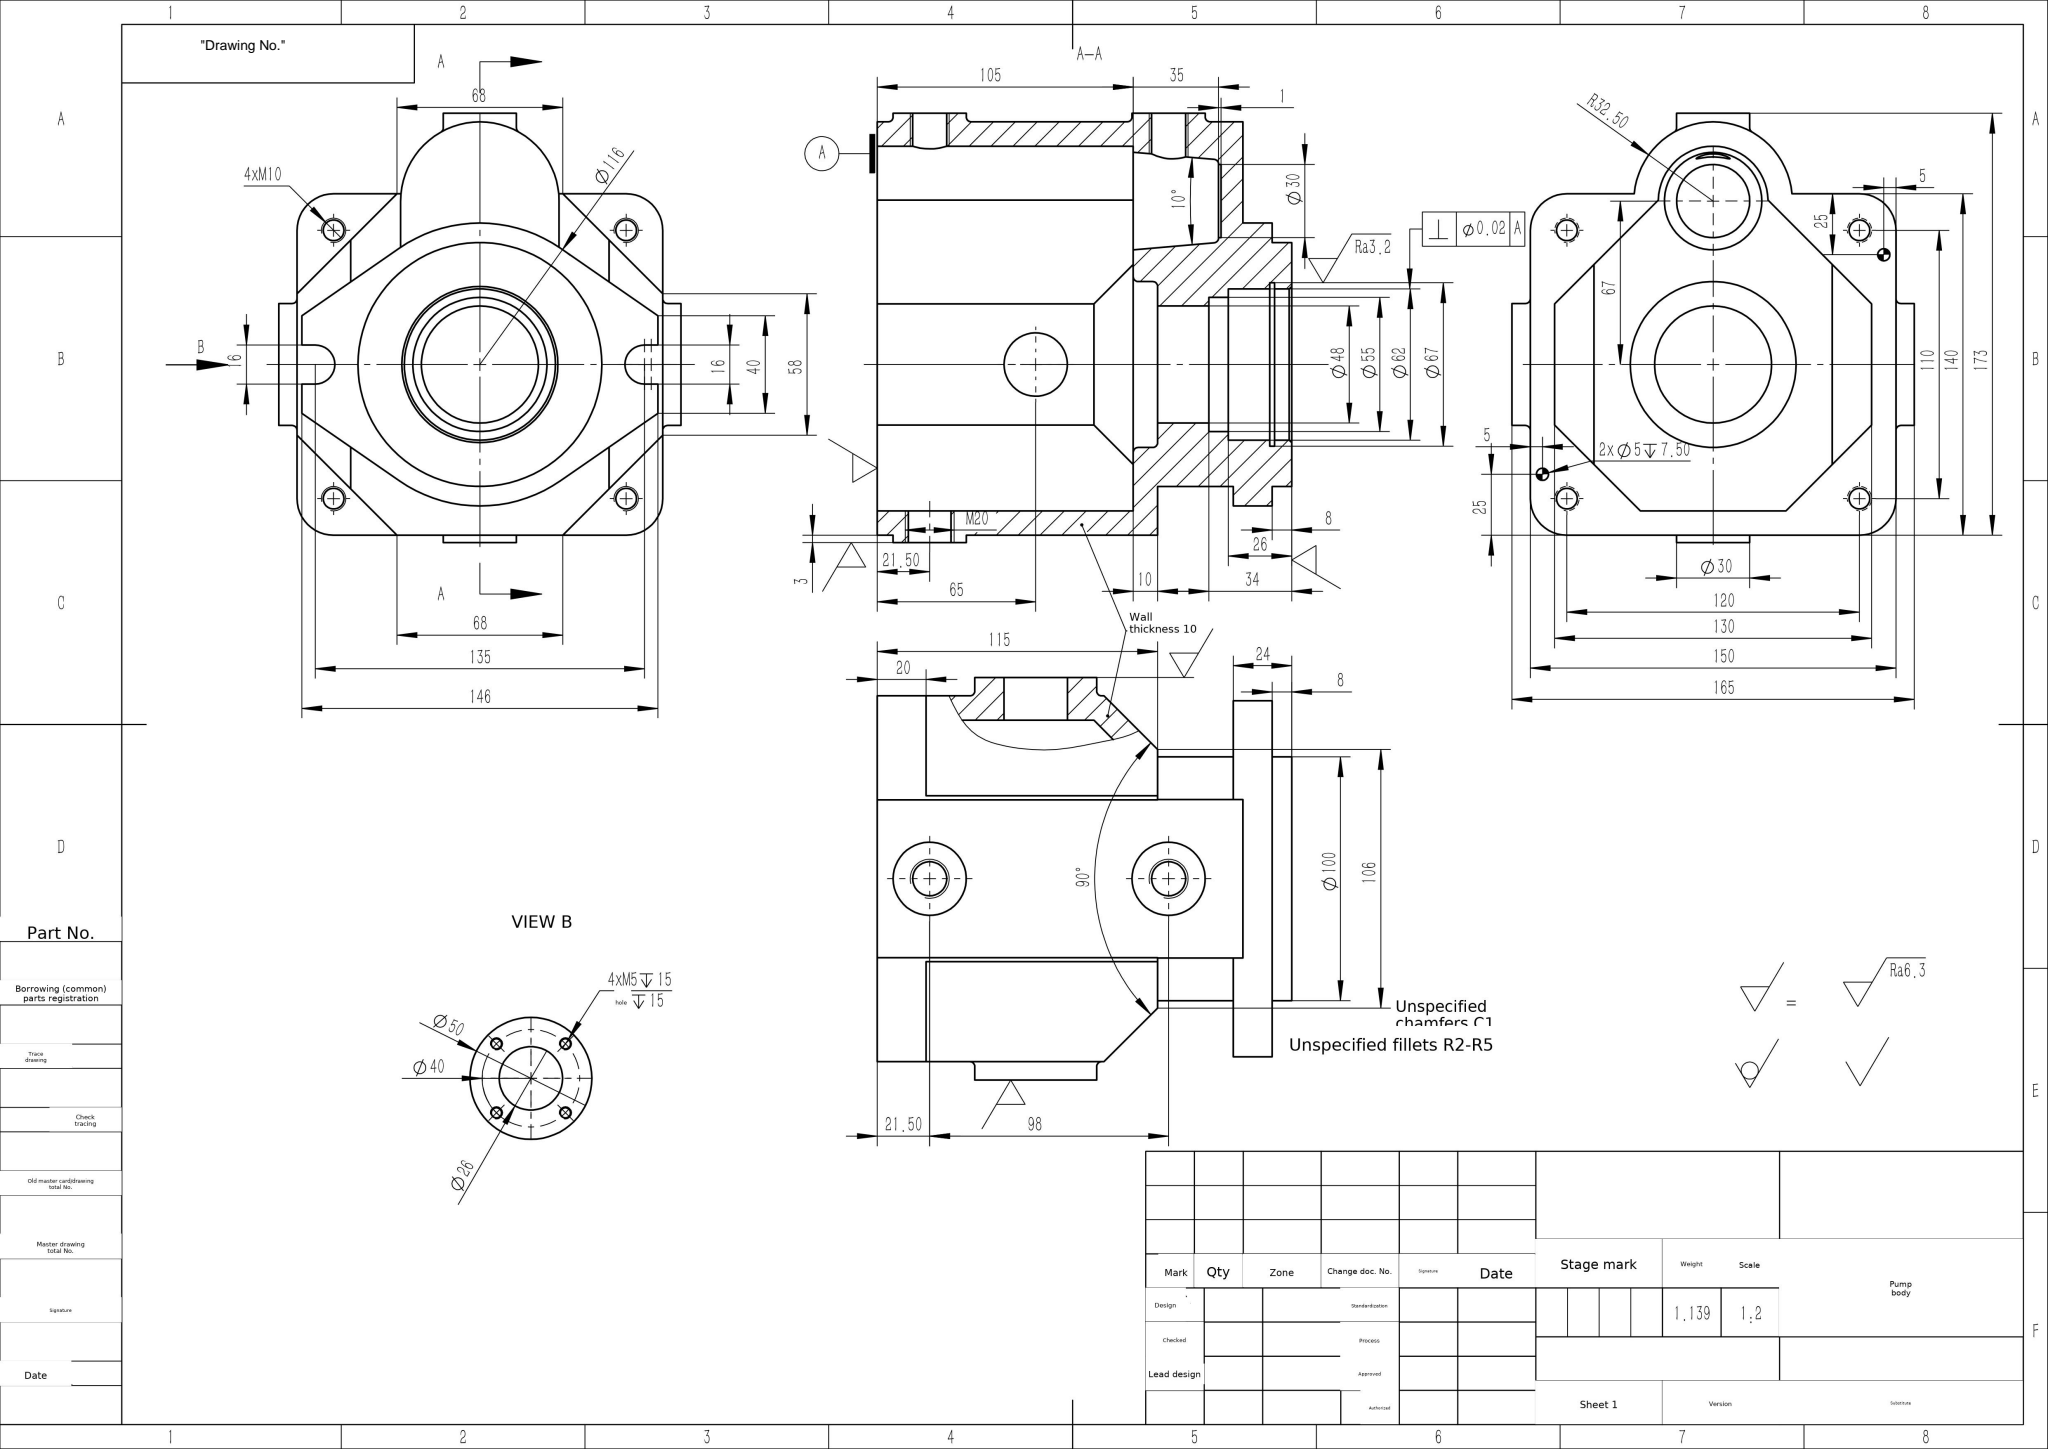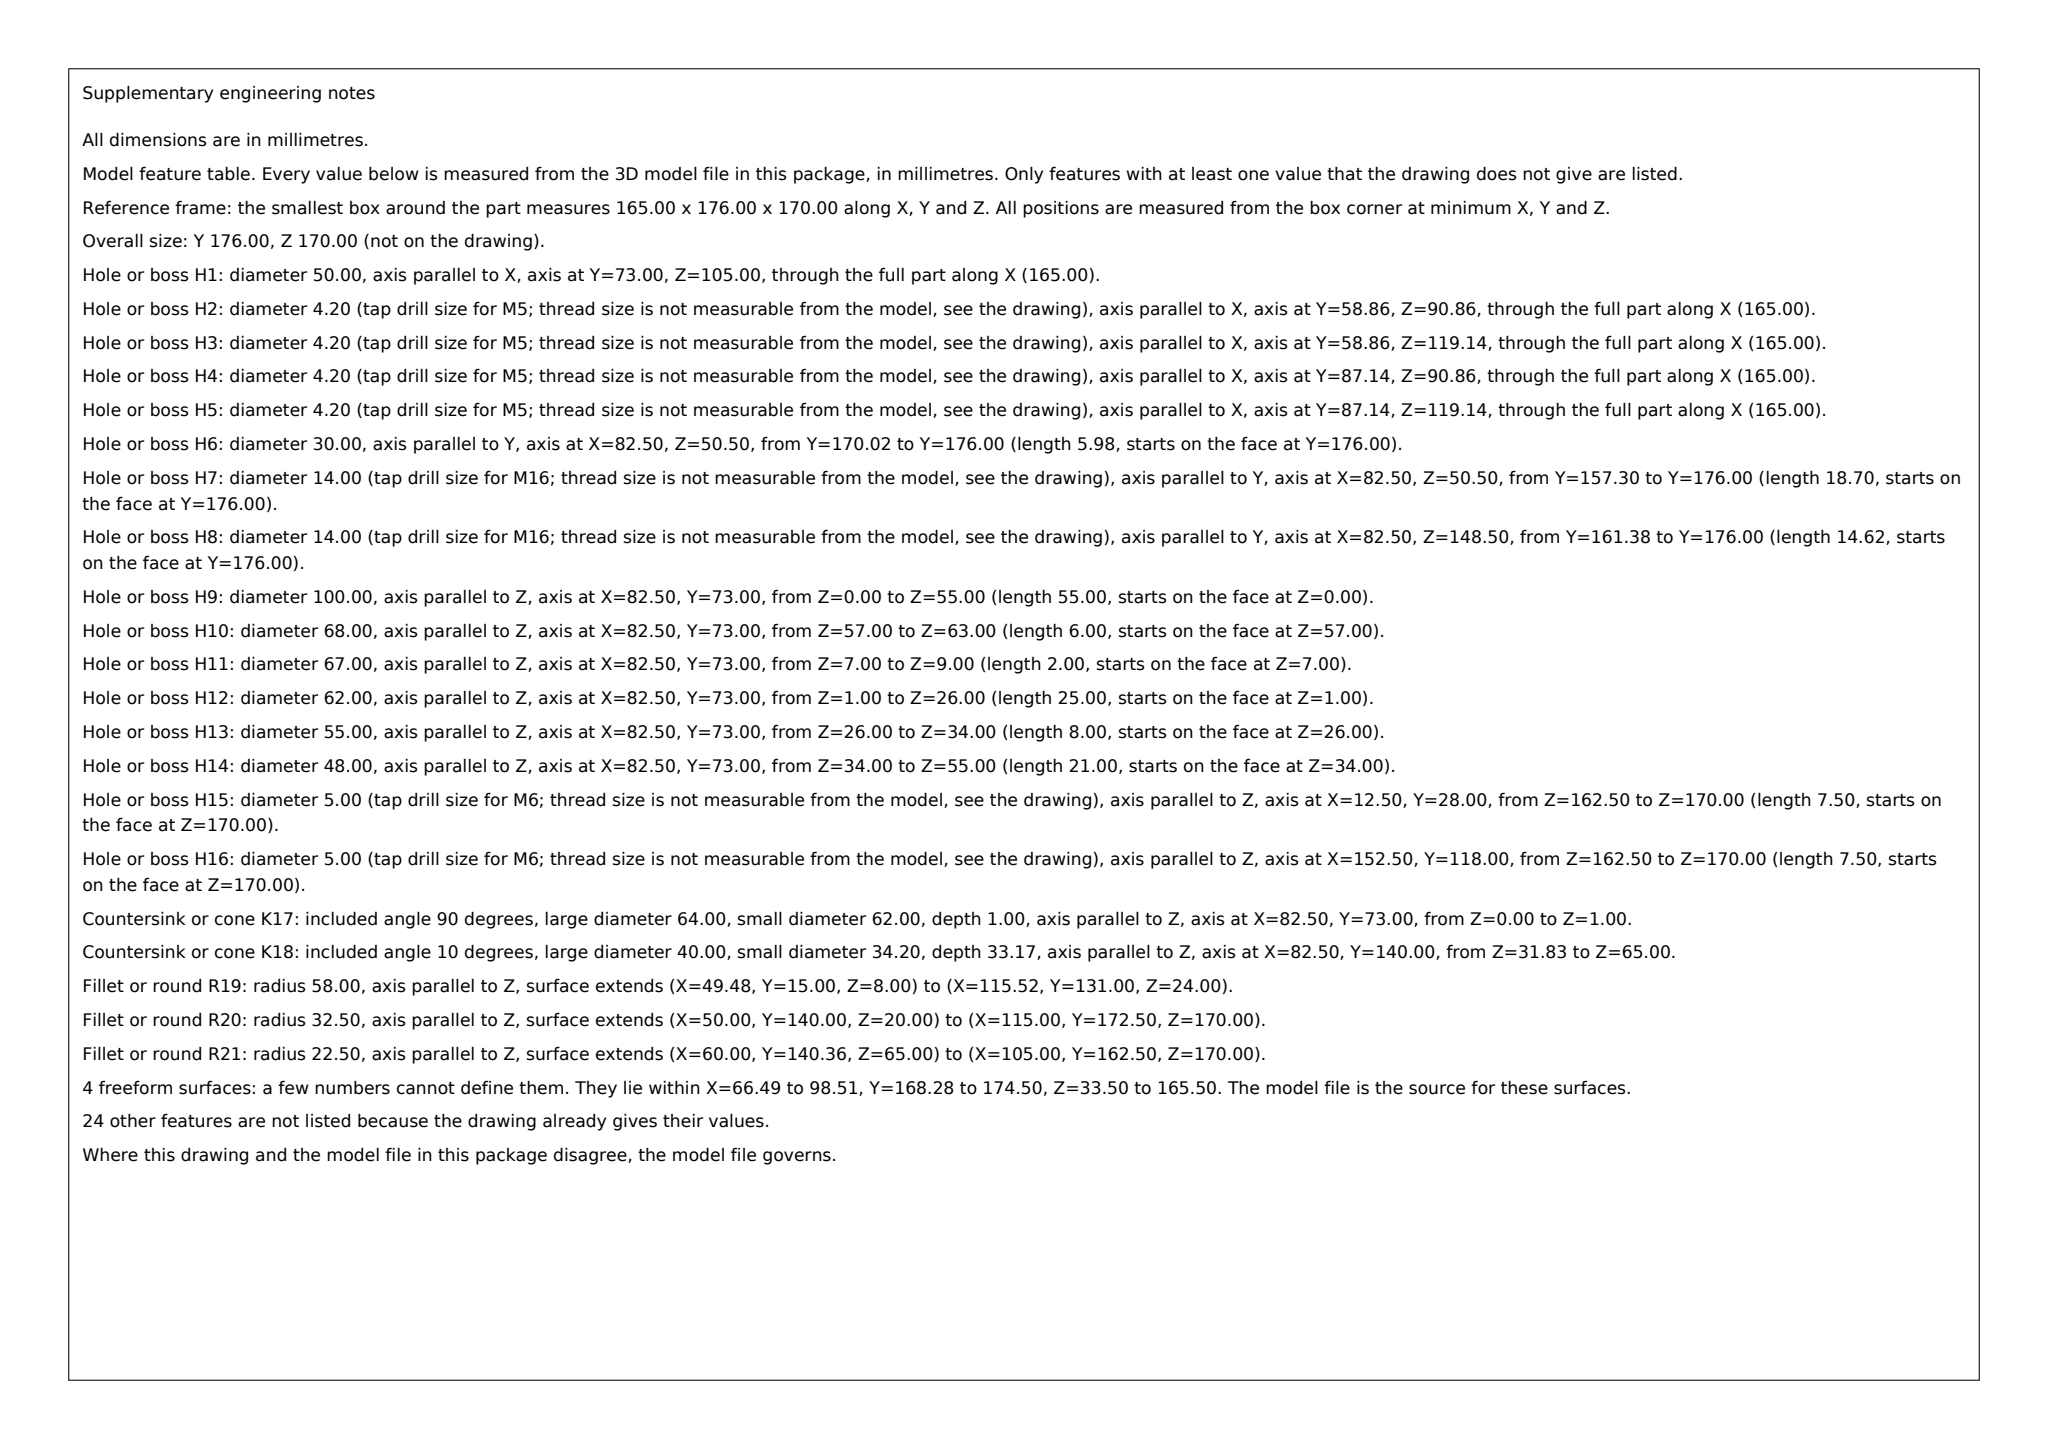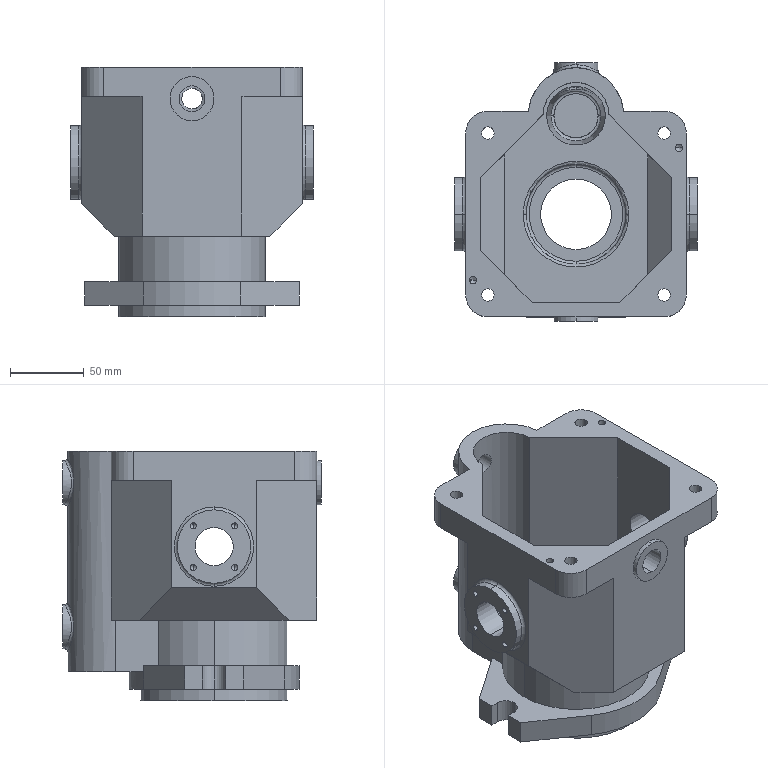Part | SolidWorks | mm | 1 solid | 173 faces | box 165 x 176 x 170 mm | volume 1139291 mm3 | cylinder 78 | plane 57 | cone 24 | torus 10 | spline 4 | commonest cylinder face diameters 4.2 x16 30 x12 8.5 x8 100 x5 5 x4 26 x4 14 x4 62 x4